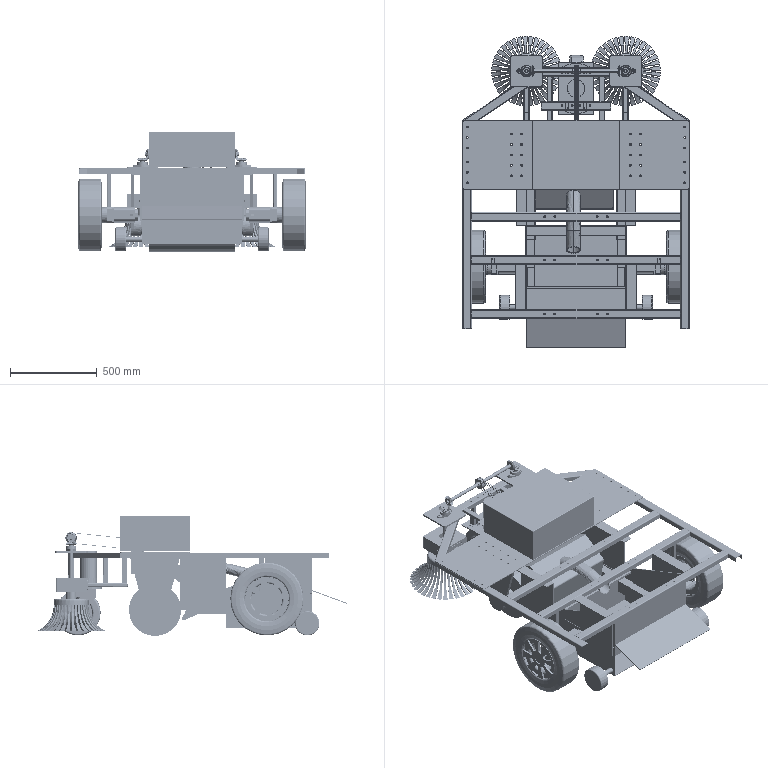Assembly | SolidWorks | mm | 97 component files | 112 solids | 5855 faces | box 1311.42 x 1789.13 x 690 mm | volume 111930544 mm3 | plane 2764 | cylinder 2030 | spline 471 | cone 310 | torus 276 | sphere 4 | commonest cylinder face diameters 10 x469 6 x221 2 x208 4 x158 8 x88 20 x80 1 x65 5 x37
Bill of materials:
50x30x2ColdBentEqualAngleSteel1000mm | 2 |  | Long, slender U-channel (formed-sheet-style profile) with a row of small round holes through the web near one end.
50x30x2ColdBentEqualAngleSteel1200mm | 4 |  | Long, slender U-channel with two pairs of small round holes in the web near the middle of its length.
50x30x2ColdBentEqualAngleSteel400 | 2 |  | Shorter U-channel with four round holes in the web and a rectangular window cut through each side flange near each end.
50x30x2ColdBentEqualAngleSteel500mm | 1 |  | Long bent strip with an angle-like profile: a flat web with a bent flange along its length and short offset or tab sections at the ends.
50x30x2ColdBentEqualAngleSteel550mmRight | 1 |  | Thin square plate with rounded corners and one central round hole. Some views also show a long, narrow channel-like strip attached to or overlapping the plate.
A30x20x2RectangularColdBentHollowSectionSteel175mm | 6 |  | Straight length of hollow rectangular tube with rounded corners, open at both ends.
A30x20x2RectangularColdFormedHollowSectionSteel220 | 2 |  | Straight length of hollow rectangular tube with rounded corners, open at both ends. It closely resembles the previous tube part.
A30x20x2RectangularColdFormedHollowSectionSteel250mm | 2 |  | Straight hollow rectangular tube with rounded corners, shown lying horizontally. The section is wider than it is tall.
Belt | 3 |  | Very thin-walled closed loop shaped like an elongated obround (stadium), similar to a band or strip loop.
BevelGear32x2 | 4 |  | Straight-tooth bevel gear with a central round bore and a single keyway.
BrushRoller | 1 |  | Stepped solid cylinder: a large-diameter central body with a smaller coaxial journal or stub shaft at each end, similar to a roller.
BrushRollerHolder | 2 |  | Hanger-type bracket: a rectangular flat top plate with a 2x5 pattern of holes, a single tapered web plate hanging below it, and a short cylindrical sleeve at the narrow lower end.
CBTCB-204.stp | 2 |  | Two-hole diamond-shaped flange with a raised round housing in the middle. A smaller cylindrical collar with a through-bore sticks up from the housing, and the collar has small radial holes.
30x20x2RectangularColdBentHollowSectionSteel900MM | 1 |  | Long straight hollow tube with a rectangular cross-section and rounded corners. One face has four small round holes, arranged as two pairs near each end.
A30x20x2RectangularColdFormedHollowSectionSteel300mm | 2 |  | Straight hollow rectangular tube fixed square to a flat rectangular plate. The plate has rounded corners and four corner holes, and the tube's opening passes through the plate.
CleaningBrush | 2 |  | Rotationally symmetric part. A small cylindrical pin with a central hole sits on top of a round hub. Many thin strip-like segments flare outward and downward from the hub in a bell or skirt shape.
CleaningBrushFixingPlate | 2 |  | Thin-walled U-shaped bracket. The flat rectangular base has four holes. Two upright side flanges are tapered, roughly triangular with a rounded tip, and each has three holes.
FixingBlock | 2 |  | Square block with rounded vertical corners. A stepped round bore goes all the way through it: a larger counterbore at the top and a smaller through-hole below. Small holes are visible on one side face.
RectangularTubeKit | 2 |  | Solid block shaped like an L (90-degree elbow), with a uniform rectangular cross-section and rounded or chamfered edges.
DriveAxis | 1 |  | Plain cylindrical shaft with chamfered ends. A short rounded-end slot (keyway) is cut into the surface near each end, both on the same side.
DriveShaft | 2 |  | Plain solid cylindrical rod or pin with flat ends and no visible features.
DriveWheel | 1 |  | Grooved wheel with three V-section grooves around its circumference. The centre bore has a keyway, and there is a recessed hub area on the face.
DSEM-GDCServoGearMotor | 1 |  | Plain cylindrical body. A small boss and a narrow shaft stick out from one end face, and the shaft has a small flat or slot.
FrontWheel | 1 |  | Wheel with a rounded tyre-like outer rim, a recessed inner face and a central hub with a small bore. Thin radial spokes or ribs connect the hub to the rim.
FrontWheelAccessory1 | 1 |  | Flat rectangular plate with a second thin layer on top that has one curved (arc) edge. A short cylindrical boss with a central hole sits on top, and small through-holes are spread across the plate.
FrontWheelAccessory2 | 1 |  | Circular disc cap with a shallow raised rim on top. Two parallel flat tabs extend down from its underside, angled to one side, and each tab ends in a rounded tip with a round hole.
GearedMotor | 1 |  | Detailed model that looks like an electric motor joined to a right-angle gearbox housing. It has a ribbed cylindrical body, a rectangular box on top with a cylindrical side spigot, a domed end cover, and a ribbed housing at the far end with a hollow bore that has a keyway.
Guard | 1 |  | Plain solid rectangular block with no visible holes or other features.
Hub | 2 |  | Spool or reel shape: a hollow cylindrical drum with a flange at each end. Inside, a spoked web has 8 openings and a small central hole.
MotorFixingPlate | 1 |  | Long, thin rectangular plate with slightly rounded corners and many small through-holes: a row along each short edge and two groups of holes in the interior.
MotorMount | 2 |  | Bent sheet-like bracket with a C-shaped profile and unequal flanges. The short top flange has 4 holes. The vertical web has a large central hole surrounded by 6 small holes on a circle. The longer bottom flange is plain.
MotorPulley1 | 1 |  | Plain cylindrical tube or spacer with a concentric through-bore and flat ends.
MotorReducer | 2 |  | Looks like a gearhead or reducer: a square front flange with 4 corner holes, a protruding round shaft, a stepped cylindrical body, and a square rear block with chamfered corners, a circular recess and a central bore.
MotorTireMotor | 2 |  | Looks like a motor body: square cross-section with cut-away corner channels, a square front flange with rounded corners and 4 holes, a round output shaft, a cylindrical rear cap, and a small block-like bump near the rear underside.
Poly-VPulley | 1 |  | Multi-groove pulley with 3 V-shaped grooves on the rim, a cylindrical hub sticking out on both sides, a central bore, a recessed face, and a small radial hole in the hub.
PushPlate | 1 |  | Thin flat rectangular plate or strip with no holes or other features.
SuctionPort | 1 |  | Prismatic block whose end profile is an irregular polygon with one large concave circular-arc edge. A bent, hollow round tube is attached to one face.
SynchronousAxis | 1 |  | Long, slender cylindrical rod with a small flat or notch near each end.
Telescopic1 | 2 |  | Straight thin-walled rectangular hollow tube with open ends.
Telescopic2 | 2 |  | Straight rectangular hollow tube with open ends and a noticeably thicker wall than a thin-gauge section.
Telescopic3 | 2 |  | Solid straight rectangular bar (a plain cuboid).
ThreadedConnectionPlate | 12 |  | L-shaped bent sheet bracket with one round through-hole in each leg.
Tire | 2 |  | Annular ring with rounded outer edges and a stepped or recessed inner face around the bore.
TorqueMotor | 2 |  | Body made of a square-section prism and a coaxial cylindrical section, with a small cylindrical shaft sticking out of the cylindrical end.
TrackPlate | 4 |  | Thin flat panel with a short bent flange along its top edge and a narrow raised line or bead across its face near the bottom.
TrashCan | 1 |  | Open-top sheet-metal box or tray with a sloped top edge on its sidewalls and rectangular cutouts. A round rod passes through it and sticks out on both sides.
TrashCanDoor | 1 |  | Thin, flat, plain rectangular plate.
TrashCanWheel | 2 |  | Thick cylindrical disc with a small central through-hole and rounded or chamfered edges.
Mates:
1. distance | 50x30x2ColdBentEqualAngleSteel1200mm-1 face at (625.629, -247.9, 410) dir (0, 1, 0) | 50x30x2ColdBentEqualAngleSteel400-1 face at (225.629, 52.1, 410) dir (0, 1, 0)
2. coincident | 50x30x2ColdBentEqualAngleSteel400-1 face at (225.629, 7.1, 415) dir (0, 0, 1) | 50x30x2ColdBentEqualAngleSteel1200mm-1 face at (625.629, -292.9, 415) dir (0, 0, 1)
3. coincident | 50x30x2ColdBentEqualAngleSteel1200mm-1 face at (-574.371, -252.9, 410) dir (-1, 0, 0) | 50x30x2ColdBentEqualAngleSteel1000mm-1 face at (-574.371, -1447.9, 410) dir (1, 0, 0)
4. coincident | 50x30x2ColdBentEqualAngleSteel1200mm-1 face at (625.629, -292.9, 415) dir (0, 0, 1) | 50x30x2ColdBentEqualAngleSteel1000mm-1 face at (-619.371, -1447.9, 415) dir (0, 0, 1)
5. coincident | 50x30x2ColdBentEqualAngleSteel1200mm-1 face at (625.629, -247.9, 410) dir (0, 1, 0) | 50x30x2ColdBentEqualAngleSteel1000mm-1 face at (-579.371, -247.9, 410) dir (0, 1, 0)
6. coincident | 50x30x2ColdBentEqualAngleSteel1200mm-1 face at (625.629, -252.9, 410) dir (1, 0, 0) | 50x30x2ColdBentEqualAngleSteel1000mm-2 face at (625.629, -1447.9, 410) dir (-1, 0, 0)
7. coincident | 50x30x2ColdBentEqualAngleSteel1200mm-1 face at (625.629, -292.9, 415) dir (0, 0, 1) | 50x30x2ColdBentEqualAngleSteel1000mm-2 face at (630.629, -1447.9, 415) dir (0, 0, 1)
8. coincident | 50x30x2ColdBentEqualAngleSteel1200mm-1 face at (625.629, -247.9, 410) dir (0, 1, 0) | 50x30x2ColdBentEqualAngleSteel1000mm-2 face at (670.629, -247.9, 410) dir (0, 1, 0)
9. coincident | 50x30x2ColdBentEqualAngleSteel400-1 face at (225.629, 7.1, 415) dir (0, 0, 1) | 50x30x2ColdBentEqualAngleSteel500mm-1 face at (-149.409, 14.658, 415) dir (0, 0, 1)
10. coincident | 50x30x2ColdBentEqualAngleSteel1000mm-1 edge at (-624.371, -247.9, 410) dir (0, 0, -1) | 50x30x2ColdBentEqualAngleSteel500mm-1 face at (-174.371, 52.1, 410) dir (-0.5547, 0.8321, 0)
11. parallel | 50x30x2ColdBentEqualAngleSteel1200mm-1 face at (625.629, -292.9, 415) dir (0, 0, 1) | CleaningRobotAssembly-1/30x20x2RectangularColdBentHollowSectionSteel900MM-2 face at (-274.371, -272.9, 238) dir (0, 0, 1)
12. coincident | 50x30x2ColdBentEqualAngleSteel400-1 edge at (-174.371, 52.1, 385) dir (0, 0, 1) | 50x30x2ColdBentEqualAngleSteel500mm-1 edge at (-174.371, 52.1, 385) dir (0, 0, 1)
13. coincident | 50x30x2ColdBentEqualAngleSteel500mm-1 face at (-149.409, 14.658, 415) dir (0, 0, 1) | 50x30x2ColdBentEqualAngleSteel550mmRight-1 face at (658.295, -290.428, 415) dir (0, 0, 1)
14. coincident | 50x30x2ColdBentEqualAngleSteel1000mm-2 edge at (675.629, -247.9, 385) dir (0, 0, 1) | 50x30x2ColdBentEqualAngleSteel550mmRight-1 face at (683.257, -252.985, 410) dir (0.5547, 0.8321, 0)
15. coincident | 50x30x2ColdBentEqualAngleSteel400-1 edge at (225.629, 52.1, 385) dir (0, 0, 1) | 50x30x2ColdBentEqualAngleSteel550mmRight-1 edge at (225.629, 52.1, 385) dir (0, 0, 1)
16. parallel | 50x30x2ColdBentEqualAngleSteel400-1 face at (225.629, 7.1, 413) dir (0, 0, -1) | FrontWheelAssembly-1/FrontWheelAccessory1-1 face at (25.629, -64.9, 238) dir (0, 0, 1)
17. parallel | 50x30x2ColdBentEqualAngleSteel400-1 face at (225.629, 7.1, 415) dir (0, 0, 1) | FrontWheelAssembly-1/FrontWheelAccessory1-1 face at (25.629, -64.9, 238) dir (0, 0, 1)
18. concentric | FrontWheelAssembly-1/FrontWheelAccessory1-1 face at (25.629, -64.9, 235) dir (0, 0, 1) r 10 | DSEM-GDCServoGearMotor-1 face at (25.629, -64.9, 232.831) dir (0, 0, -1) r 7
19. coincident | FrontWheelAssembly-1/FrontWheelAccessory1-1 face at (25.629, -64.9, 268) dir (0, 0, 1) | DSEM-GDCServoGearMotor-1 face at (44.794, -59.181, 268) dir (0, 0, -1)
20. parallel | 50x30x2ColdBentEqualAngleSteel1000mm-1 face at (-624.371, -1447.9, 410) dir (-1, 0, 0) | FrontWheelAssembly-1/FrontWheelAccessory1-1 face at (-74.371, -214.9, 233) dir (-1, 0, 0)
21. coincident | 50x30x2ColdBentEqualAngleSteel400-1 face at (225.629, 7.1, 413) dir (0, 0, -1) | A30x20x2RectangularColdBentHollowSectionSteel175mm-1 face at (76.629, 35.1, 413) dir (0, 0, 1)
22. parallel | 50x30x2ColdBentEqualAngleSteel400-1 face at (225.629, 52.1, 410) dir (0, 1, 0) | A30x20x2RectangularColdBentHollowSectionSteel175mm-1 face at (76.629, 50.1, 238) dir (0, 1, 0)
23. coincident | 50x30x2ColdBentEqualAngleSteel400-1 face at (225.629, 50.1, 410) dir (0, -1, 0) | A30x20x2RectangularColdBentHollowSectionSteel175mm-1 face at (76.629, 50.1, 238) dir (0, 1, 0)
24. coincident | FrontWheelAssembly-1/FrontWheelAccessory1-1 face at (25.629, -64.9, 238) dir (0, 0, 1) | A30x20x2RectangularColdBentHollowSectionSteel175mm-1 face at (76.629, 35.1, 238) dir (0, 0, -1)
25. coincident | FrontWheelAssembly-1/FrontWheelAccessory1-1 face at (25.629, -64.9, 238) dir (0, 0, 1) | ThreadedConnectionPlate-1 face at (102.629, 35.1, 238) dir (0, 0, -1)
26. coincident | A30x20x2RectangularColdBentHollowSectionSteel175mm-1 face at (86.629, 35.1, 238) dir (1, 0, 0) | ThreadedConnectionPlate-1 face at (86.629, 35.1, 238) dir (-1, 0, 0)
27. coincident | A30x20x2RectangularColdBentHollowSectionSteel175mm-1 face at (76.629, 50.1, 238) dir (0, 1, 0) | ThreadedConnectionPlate-1 face at (117.629, 50.1, 239) dir (0, 1, 0)
28. concentric | FrontWheelAssembly-1/FrontWheelAccessory1-1 face at (105.629, 35.1, 238) dir (0, 0, -1) r 5 | ThreadedConnectionPlate-1 face at (105.629, 35.1, 238) dir (0, 0, 1) r 5
29. coincident | A30x20x2RectangularColdBentHollowSectionSteel175mm-1 face at (66.629, 35.1, 238) dir (-1, 0, 0) | ThreadedConnectionPlate-6 face at (66.629, 35.1, 238) dir (1, 0, 0)
30. coincident | A30x20x2RectangularColdBentHollowSectionSteel175mm-1 face at (76.629, 50.1, 238) dir (0, 1, 0) | ThreadedConnectionPlate-6 face at (35.629, 50.1, 239) dir (0, 1, 0)
31. coincident | FrontWheelAssembly-1/FrontWheelAccessory1-1 face at (25.629, -64.9, 238) dir (0, 0, 1) | ThreadedConnectionPlate-6 face at (50.629, 35.1, 238) dir (0, 0, -1)
32. coincident | 50x30x2ColdBentEqualAngleSteel400-1 face at (225.629, 7.1, 413) dir (0, 0, -1) | A30x20x2RectangularColdBentHollowSectionSteel175mm-4 face at (-25.371, 35.1, 413) dir (0, 0, 1)
33. coincident | 50x30x2ColdBentEqualAngleSteel400-1 face at (225.629, 50.1, 410) dir (0, -1, 0) | A30x20x2RectangularColdBentHollowSectionSteel175mm-4 face at (-25.371, 50.1, 238) dir (0, 1, 0)
34. coincident | FrontWheelAssembly-1/FrontWheelAccessory1-1 face at (25.629, -64.9, 238) dir (0, 0, 1) | ThreadedConnectionPlate-10 face at (0.6293, 35.1, 238) dir (0, 0, -1)
35. coincident | ThreadedConnectionPlate-10 face at (-15.371, 35.1, 238) dir (-1, 0, 0) | A30x20x2RectangularColdBentHollowSectionSteel175mm-4 face at (-15.371, 35.1, 238) dir (1, 0, 0)
36. concentric | FrontWheelAssembly-1/FrontWheelAccessory1-1 face at (3.629, 35.1, 253) dir (0, 0, -1) r 5.507 | ThreadedConnectionPlate-10 face at (3.629, 35.1, 238) dir (0, 0, 1) r 5
37. concentric | FrontWheelAssembly-1/FrontWheelAccessory1-1 face at (-54.371, 35.1, 238) dir (0, 0, -1) r 5 | ThreadedConnectionPlate-8 face at (-54.371, 35.1, 238) dir (0, 0, 1) r 5
38. coincident | FrontWheelAssembly-1/FrontWheelAccessory1-1 face at (25.629, -64.9, 238) dir (0, 0, 1) | ThreadedConnectionPlate-8 face at (-51.371, 35.1, 238) dir (0, 0, -1)
39. coincident | ThreadedConnectionPlate-8 face at (-35.371, 35.1, 238) dir (1, 0, 0) | A30x20x2RectangularColdBentHollowSectionSteel175mm-4 face at (-35.371, 35.1, 238) dir (-1, 0, 0)
40. coincident | A30x20x2RectangularColdBentHollowSectionSteel175mm-3 face at (76.629, -164.9, 413) dir (0, 0, 1) | 50x30x2ColdBentEqualAngleSteel400-2 face at (225.629, -184.9, 413) dir (0, 0, -1)
41. coincident | 50x30x2ColdBentEqualAngleSteel400-1 face at (-174.371, 47.1, 410) dir (-1, 0, 0) | 50x30x2ColdBentEqualAngleSteel400-2 face at (-174.371, -144.9, 410) dir (-1, 0, 0)
42. coincident | 50x30x2ColdBentEqualAngleSteel1200mm-1 face at (625.629, -247.9, 410) dir (0, 1, 0) | A30x20x2RectangularColdFormedHollowSectionSteel250mm-1 face at (-124.591, -247.9, 400) dir (0, -1, 0)
43. distance | A30x20x2RectangularColdFormedHollowSectionSteel250mm-1 face at (-124.591, -247.9, 410) dir (0, 0, 1) | 50x30x2ColdBentEqualAngleSteel400-1 face at (225.629, 7.1, 415) dir (0, 0, 1)
44. coincident | 50x30x2ColdBentEqualAngleSteel400-1 face at (185.629, -14.9, 410) dir (0, 0, -1) | A30x20x2RectangularColdFormedHollowSectionSteel250mm-2 face at (175.629, -247.9, 410) dir (0, 0, 1)
45. coincident | 50x30x2ColdBentEqualAngleSteel400-1 face at (160.629, -14.9, 395) dir (1, 0, 0) | A30x20x2RectangularColdFormedHollowSectionSteel250mm-2 face at (160.629, -247.9, 400) dir (-1, 0, 0)
46. coincident | 50x30x2ColdBentEqualAngleSteel400-1 face at (225.629, 52.1, 410) dir (0, 1, 0) | A30x20x2RectangularColdFormedHollowSectionSteel250mm-2 face at (175.629, 52.1, 400) dir (0, 1, 0)
47. concentric | FrontWheelAssembly-1/FrontWheelAccessory1-1 face at (-54.371, -164.9, 144) dir (0, 0, 1) r 5 | 50x30x2ColdBentEqualAngleSteel400-2 face at (-54.371, -164.9, 350) dir (0, 0, 1) r 5
48. coincident | CleaningRobotAssembly-1/30x20x2RectangularColdBentHollowSectionSteel900MM-2 face at (-274.371, -272.9, 238) dir (0, 0, 1) | A30x20x2RectangularColdBentHollowSectionSteel175mm-6 face at (176.629, -272.9, 238) dir (0, 0, -1)
49. coincident | 50x30x2ColdBentEqualAngleSteel1200mm-1 face at (625.629, -292.9, 413) dir (0, 0, -1) | A30x20x2RectangularColdBentHollowSectionSteel175mm-6 face at (176.629, -272.9, 413) dir (0, 0, 1)
50. coincident | A30x20x2RectangularColdBentHollowSectionSteel175mm-6 face at (186.629, -272.9, 238) dir (1, 0, 0) | ThreadedConnectionPlate-12 face at (186.629, -272.9, 238) dir (-1, 0, 0)
51. coincident | A30x20x2RectangularColdBentHollowSectionSteel175mm-6 face at (176.629, -287.9, 238) dir (0, -1, 0) | ThreadedConnectionPlate-12 face at (217.629, -287.9, 239) dir (0, -1, 0)
52. concentric | CleaningRobotAssembly-1/30x20x2RectangularColdBentHollowSectionSteel900MM-2 face at (205.629, -272.9, 301) dir (0, 0, -1) r 5 | ThreadedConnectionPlate-12 face at (205.629, -272.9, 238) dir (0, 0, 1) r 5
53. coincident | CleaningRobotAssembly-1/30x20x2RectangularColdBentHollowSectionSteel900MM-2 face at (-274.371, -272.9, 238) dir (0, 0, 1) | ThreadedConnectionPlate-12 face at (202.629, -272.9, 238) dir (0, 0, -1)
54. concentric | CleaningRobotAssembly-1/30x20x2RectangularColdBentHollowSectionSteel900MM-2 face at (147.629, -272.9, 301) dir (0, 0, -1) r 5 | ThreadedConnectionPlate-13 face at (147.629, -272.9, 238) dir (0, 0, 1) r 5
55. coincident | CleaningRobotAssembly-1/30x20x2RectangularColdBentHollowSectionSteel900MM-2 face at (-274.371, -272.9, 238) dir (0, 0, 1) | ThreadedConnectionPlate-13 face at (150.629, -272.9, 238) dir (0, 0, -1)
56. coincident | A30x20x2RectangularColdBentHollowSectionSteel175mm-6 face at (166.629, -272.9, 238) dir (-1, 0, 0) | ThreadedConnectionPlate-13 face at (166.629, -272.9, 238) dir (1, 0, 0)
57. coincident | 50x30x2ColdBentEqualAngleSteel1000mm-1 face at (-624.371, -1447.9, 410) dir (-1, 0, 0) | MotorFixingPlate-1 face at (-624.371, -647.9, 420) dir (-1, 0, 0)
58. coincident | 50x30x2ColdBentEqualAngleSteel1000mm-1 face at (-619.371, -1447.9, 415) dir (0, 0, 1) | MotorFixingPlate-1 face at (25.629, -447.9, 415) dir (0, 0, -1)
59. parallel | MotorFixingPlate-1 face at (25.629, -447.9, 415) dir (0, 0, -1) | TorqueMotor-1 face at (-92.371, -325.407, 376) dir (0, 0, 1)
60. concentric | BrushRoller-1 face at (-324.371, -447.9, 85) dir (1, 0, 0) r 50 | BrushRollerHolder-1 face at (-308.371, -447.9, 85) dir (-1, 0, 0) r 50
61. coincident | MotorFixingPlate-1 face at (25.629, -447.9, 415) dir (0, 0, -1) | BrushRollerHolder-1 face at (-316.371, -447.9, 415) dir (0, 0, 1)
62. concentric | MotorFixingPlate-1 face at (-345.371, -567.9, 380) dir (0, 0, 1) r 5 | BrushRollerHolder-1 face at (-345.371, -567.9, 450) dir (0, 0, -1) r 5
63. coincident | MotorFixingPlate-1 face at (25.629, -447.9, 415) dir (0, 0, -1) | MotorMount-1 face at (-227.371, -367.407, 415) dir (0, 0, 1)
64. concentric | TorqueMotor-1 face at (-224.371, -367.407, 334) dir (1, 0, 0) r 37 | MotorMount-1 face at (-248.371, -367.407, 334) dir (1, 0, 0) r 20
65. concentric | TorqueMotor-1 face at (-214.371, -367.407, 364) dir (-1, 0, 0) r 3 | MotorMount-1 face at (-224.371, -367.407, 364) dir (-1, 0, 0) r 3
66. coincident | TorqueMotor-1 face at (-224.371, -367.407, 334) dir (-1, 0, 0) | MotorMount-1 face at (-224.371, -367.407, 334) dir (1, 0, 0)
67. concentric | MotorFixingPlate-1 face at (-287.371, -567.9, 380) dir (0, 0, 1) r 5 | BrushRollerHolder-1 face at (-287.371, -567.9, 450) dir (0, 0, -1) r 5
68. concentric | TorqueMotor-1 face at (-254.371, -367.407, 334) dir (1, 0, 0) r 8 | MotorPulley1-1 face at (-234.371, -367.407, 334) dir (-1, 0, 0) r 8
69. coincident | TorqueMotor-1 face at (-254.371, -367.407, 334) dir (-1, 0, 0) | MotorPulley1-1 face at (-254.371, -367.407, 334) dir (-1, 0, 0)
70. concentric | MotorTireMotor-1 face at (-468.371, -1090.9, 148) dir (1, 0, 0) r 11 | MotorReducer-1 face at (-470.371, -1090.9, 148) dir (1, 0, 0) r 11
71. coincident | MotorTireMotor-1 face at (-434.371, -1090.9, 148) dir (-1, 0, 0) | MotorReducer-1 face at (-434.371, -1090.9, 148) dir (1, 0, 0)
72. coincident | MotorTireMotor-1 face at (-422.371, -1045.9, 193) dir (0, 0, 1) | MotorReducer-1 face at (-462.371, -1135.9, 193) dir (0, 0, 1)
73. concentric | Hub-1 face at (-621.371, -1090.9, 148) dir (-1, 0, 0) r 93 | Tire-1 face at (-664.825, -1090.9, 148) dir (-1, 0, 0) r 108
74. coincident | Hub-1 face at (-608.371, -1009.58, 206.198) dir (1, 0, 0) | Tire-1 face at (-608.371, -983.391, 137.711) dir (-1, 0, 0)
75. concentric | Hub-1 face at (-501.371, -1090.9, 148) dir (-1, 0, 0) r 10 | MotorReducer-1 face at (-619.371, -1090.9, 148) dir (1, 0, 0) r 10
76. coincident | Hub-1 face at (-619.371, -1090.9, 148) dir (-1, 0, 0) | MotorReducer-1 face at (-619.371, -1090.9, 148) dir (-1, 0, 0)
77. coincident | 50x30x2ColdBentEqualAngleSteel1000mm-1 face at (-574.371, -1447.9, 410) dir (1, 0, 0) | 50x30x2ColdBentEqualAngleSteel1200mm-2 face at (-574.371, -1032.9, 410) dir (-1, 0, 0)
78. coincident | 50x30x2ColdBentEqualAngleSteel1000mm-1 face at (-619.371, -1447.9, 415) dir (0, 0, 1) | 50x30x2ColdBentEqualAngleSteel1200mm-2 face at (625.629, -1072.9, 415) dir (0, 0, 1)
79. parallel | MotorTireMotor-1 face at (-422.371, -1045.9, 193) dir (0, 0, 1) | 50x30x2ColdBentEqualAngleSteel1200mm-2 face at (625.629, -1072.9, 413) dir (0, 0, -1)
80. coincident | 50x30x2ColdBentEqualAngleSteel1200mm-2 face at (625.629, -1072.9, 413) dir (0, 0, -1) | A30x20x2RectangularColdFormedHollowSectionSteel220-1 face at (-452.371, -1060.9, 413) dir (0, 0, 1)
81. coincident | MotorReducer-1 face at (-462.371, -1135.9, 193) dir (0, 0, 1) | A30x20x2RectangularColdFormedHollowSectionSteel220-1 face at (-452.371, -1060.9, 193) dir (0, 0, -1)
82. coincident | 50x30x2ColdBentEqualAngleSteel1200mm-2 face at (625.629, -1075.9, 410) dir (0, 1, 0) | A30x20x2RectangularColdFormedHollowSectionSteel220-1 face at (-452.371, -1075.9, 413) dir (0, -1, 0)
83. coincident | MotorReducer-1 face at (-462.371, -1045.9, 103) dir (0, 1, 0) | A30x20x2RectangularColdFormedHollowSectionSteel220-1 face at (-452.371, -1045.9, 413) dir (0, 1, 0)
84. parallel | 50x30x2ColdBentEqualAngleSteel1000mm-1 face at (-579.371, -1447.9, 410) dir (0, -1, 0) | TrashCan-1 face at (-264.371, -1353.331, 103.161) dir (0, -1, 0)
85. coincident | BrushRoller-1 face at (-324.371, -447.9, 85) dir (-1, 0, 0) | BrushRollerHolder-1 face at (-324.371, -447.9, 85) dir (-1, 0, 0)
86. parallel | BrushRollerHolder-1 face at (-324.371, -447.9, 85) dir (-1, 0, 0) | MotorMount-1 face at (-227.371, -367.407, 334) dir (-1, 0, 0)
87. coincident | BrushRoller-1 face at (-224.371, -447.9, 85) dir (-1, 0, 0) | TorqueMotor-1 face at (-224.371, -367.407, 334) dir (-1, 0, 0)
88. coincident | 50x30x2ColdBentEqualAngleSteel1200mm-1 face at (625.629, -247.9, 410) dir (0, 1, 0) | MotorFixingPlate-1 face at (-624.371, -247.9, 420) dir (0, 1, 0)
89. concentric | MotorFixingPlate-1 face at (-212.371, -407.407, 895) dir (0, 0, -1) r 5 | MotorMount-1 face at (-212.371, -407.407, 412) dir (0, 0, 1) r 5
90. concentric | MotorFixingPlate-1 face at (-212.371, -327.407, 895) dir (0, 0, -1) r 5 | MotorMount-1 face at (-212.371, -327.407, 412) dir (0, 0, 1) r 5
91. coincident | 50x30x2ColdBentEqualAngleSteel1000mm-1 face at (-574.371, -1447.9, 410) dir (1, 0, 0) | 50x30x2ColdBentEqualAngleSteel1200mm-3 face at (-574.371, -1342.9, 410) dir (-1, 0, 0)
92. coincident | 50x30x2ColdBentEqualAngleSteel1000mm-1 face at (-619.371, -1447.9, 415) dir (0, 0, 1) | 50x30x2ColdBentEqualAngleSteel1200mm-3 face at (625.629, -1382.9, 415) dir (0, 0, 1)
93. distance | 50x30x2ColdBentEqualAngleSteel1200mm-2 face at (625.629, -1077.9, 410) dir (0, -1, 0) | 50x30x2ColdBentEqualAngleSteel1200mm-3 face at (625.629, -1337.9, 410) dir (0, 1, 0)
94. coincident | 50x30x2ColdBentEqualAngleSteel1000mm-1 face at (-624.371, -1447.9, 410) dir (-1, 0, 0) | Hub-1 face at (-624.371, -1090.9, 148) dir (-1, 0, 0)
95. coincident | MotorReducer-1 face at (-462.371, -1090.9, 148) dir (-1, 0, 0) | A30x20x2RectangularColdFormedHollowSectionSteel220-1 face at (-462.371, -1060.9, 413) dir (-1, 0, 0)
96. coincident | TrashCan-1 face at (-264.371, -1353.331, -21.839) dir (-1, 0, 0) | TrackPlate-1 face at (-264.371, -1337.9, 410) dir (1, 0, 0)
97. coincident | 50x30x2ColdBentEqualAngleSteel1200mm-3 face at (625.629, -1382.9, 415) dir (0, 0, 1) | TrackPlate-1 face at (-294.371, -1207.9, 415) dir (0, 0, 1)
98. coincident | 50x30x2ColdBentEqualAngleSteel1200mm-2 face at (625.629, -1077.9, 410) dir (0, -1, 0) | TrackPlate-1 face at (-264.371, -1077.9, 410) dir (0, 1, 0)
99. distance | 50x30x2ColdBentEqualAngleSteel1200mm-3 face at (625.629, -1387.9, 410) dir (0, -1, 0) | 50x30x2ColdBentEqualAngleSteel1000mm-1 face at (-579.371, -1447.9, 410) dir (0, -1, 0)
100. coincident | 50x30x2ColdBentEqualAngleSteel1200mm-2 face at (625.629, -1077.9, 410) dir (0, -1, 0) | TrackPlate-2 face at (315.629, -1077.9, 410) dir (0, 1, 0)
101. coincident | 50x30x2ColdBentEqualAngleSteel1200mm-2 face at (625.629, -1072.9, 415) dir (0, 0, 1) | TrackPlate-2 face at (345.629, -1207.9, 415) dir (0, 0, 1)
102. coincident | TrashCan-1 face at (315.629, -1353.331, -21.839) dir (1, 0, 0) | TrackPlate-2 face at (315.629, -1077.9, 410) dir (-1, 0, 0)
103. concentric | TrashCan-1 face at (-264.371, -939.331, 178.161) dir (0, -1, 0) r 2.5 | TrackPlate-1 face at (-264.371, -1070.829, 178.161) dir (0, -1, 0) r 2.5
104. parallel | 50x30x2ColdBentEqualAngleSteel1200mm-1 face at (625.629, -297.9, 410) dir (0, -1, 0) | CleaningRobotAssembly-1/RectangularTubeKit-1 face at (322.629, -289.9, 221) dir (0, -1, 0)
105. concentric | 50x30x2ColdBentEqualAngleSteel1200mm-1 face at (-154.371, -272.9, 405) dir (0, 0, 1) r 5 | CleaningRobotAssembly-1/30x20x2RectangularColdBentHollowSectionSteel900MM-2 face at (-154.371, -272.9, 301) dir (0, 0, -1) r 5
106. distance | TrackPlate-1 face at (-264.371, -1337.9, 410) dir (1, 0, 0) | 50x30x2ColdBentEqualAngleSteel1000mm-1 face at (-574.371, -1447.9, 410) dir (1, 0, 0)
107. concentric | TrashCan-1 face at (-414.371, -1323.331, 8.161) dir (1, 0, 0) r 15 | TrashCanWheel-3 face at (-414.371, -1323.331, 8.161) dir (1, 0, 0) r 15
108. coincident | TrashCan-1 face at (-414.371, -1323.331, 8.161) dir (-1, 0, 0) | TrashCanWheel-3 face at (-414.371, -1323.331, 8.161) dir (-1, 0, 0)
109. concentric | TrashCan-1 face at (465.629, -1323.331, 8.161) dir (-1, 0, 0) r 15 | TrashCanWheel-4 face at (405.629, -1323.331, 8.161) dir (1, 0, 0) r 15
110. coincident | TrashCan-1 face at (465.629, -1323.331, 8.161) dir (1, 0, 0) | TrashCanWheel-4 face at (465.629, -1323.331, 8.161) dir (1, 0, 0)
111. distance | SuctionPort-1 face at (240.629, -545.604, 83.86) dir (1, 0, 0) | TrashCan-1 face at (315.629, -1353.331, -21.839) dir (1, 0, 0)
112. coincident | SuctionPort-1 face at (-209.371, -545.604, 83.86) dir (-1, 0, 0) | Telescopic1-1 face at (-209.371, -636.122, 139.31) dir (1, 0, 0)
113. parallel | CleaningRobotAssembly-1/CleaningBrushFixingPlate-3 face at (-350.371, -57.9, 188) dir (0, -1, 0) | Telescopic1-1 face at (-234.371, -636.122, 101.81) dir (0, 1, 0)
114. coincident | Telescopic1-1 face at (-257.371, -436.122, 67.31) dir (0, 0, 1) | Telescopic2-1 face at (-257.371, -793.365, 67.31) dir (0, 0, -1)
115. coincident | Telescopic1-1 face at (-257.371, -436.122, 67.31) dir (1, 0, 0) | Telescopic2-1 face at (-257.371, -793.365, 67.31) dir (-1, 0, 0)
116. coincident | TrashCan-1 face at (-264.371, -1230.322, -16.839) dir (0, 0, 1) | PushPlate-1 face at (-259.371, -1216.787, -16.839) dir (0, 0, -1)
117. coincident | TrashCan-1 face at (310.629, -1353.331, -21.839) dir (-1, 0, 0) | PushPlate-1 face at (310.629, -1216.787, -16.839) dir (1, 0, 0)
118. coincident | Telescopic2-1 face at (-254.371, -1093.365, 72.31) dir (1, 0, 0) | Telescopic3-1 face at (-254.371, -906.787, 72.31) dir (-1, 0, 0)
119. coincident | Telescopic2-1 face at (-254.371, -1093.365, 72.31) dir (0, 0, 1) | Telescopic3-1 face at (-254.371, -906.787, 72.31) dir (0, 0, -1)
120. coincident | PushPlate-1 face at (25.629, -1206.787, 90.661) dir (0, 1, 0) | Telescopic3-1 face at (-234.371, -1206.787, 102.31) dir (0, -1, 0)
121. distance | Telescopic2-1 face at (-234.371, -1093.365, 102.31) dir (0, -1, 0) | Telescopic1-1 face at (-234.371, -936.122, 101.81) dir (0, -1, 0)
122. distance | PushPlate-1 face at (25.629, -1206.787, 90.661) dir (0, 1, 0) | Telescopic2-1 face at (-234.371, -1093.365, 102.31) dir (0, -1, 0)
123. coincident | 50x30x2ColdBentEqualAngleSteel1000mm-1 face at (-574.371, -1447.9, 410) dir (1, 0, 0) | 50x30x2ColdBentEqualAngleSteel1200mm-4 face at (-574.371, -782.9, 410) dir (-1, 0, 0)
124. coincident | 50x30x2ColdBentEqualAngleSteel1000mm-1 face at (-619.371, -1447.9, 415) dir (0, 0, 1) | 50x30x2ColdBentEqualAngleSteel1200mm-4 face at (625.629, -822.9, 415) dir (0, 0, 1)
125. distance | 50x30x2ColdBentEqualAngleSteel1200mm-4 face at (625.629, -827.9, 410) dir (0, -1, 0) | 50x30x2ColdBentEqualAngleSteel1200mm-2 face at (625.629, -1027.9, 410) dir (0, 1, 0)
126. coincident | Telescopic1-1 face at (-259.371, -636.122, 139.31) dir (-1, 0, 0) | TrackPlate-3 face at (-259.371, -853.293, 380) dir (1, 0, 0)
127. coincident | 50x30x2ColdBentEqualAngleSteel1200mm-4 face at (625.629, -777.9, 385) dir (0, 0, -1) | TrackPlate-3 face at (-289.371, -723.293, 385) dir (0, 0, 1)
128. coincident | TrashCan-1 face at (-259.371, -1353.331, -21.839) dir (1, 0, 0) | TrashCanDoor-1 face at (-259.371, -1351.6, 193.47) dir (-1, 0, 0)
129. coincident | TrashCan-1 edge at (310.629, -1353.331, 198.161) dir (-1, 0, 0) | TrashCanDoor-1 edge at (-259.371, -1353.331, 198.161) dir (1, 0, 0)
130. concentric | CleaningRobotAssembly-1/CleaningBrush-1 face at (310.629, 34.1, 198) dir (0, 0, 1) r 10 | CBTCB-204.stp-1 face at (310.629, 34.1, 436) dir (0, 0, 1) r 10
131. coincident | 50x30x2ColdBentEqualAngleSteel550mmRight-1 face at (197.894, 10.497, 425) dir (0, 0, 1) | CBTCB-204.stp-1 face at (265.629, 34.1, 425) dir (0, 0, -1)
132. parallel | CleaningRobotAssembly-1/FixingBlock-1 face at (400.629, 124.1, 188) dir (0, 1, 0) | CBTCB-204.stp-1 face at (355.629, 45.6, 434) dir (0, 1, 0)
133. concentric | CleaningRobotAssembly-1/FixingBlock-3 face at (-259.371, 34.1, 288) dir (0, 0, -1) r 32.5 | CBTCB-204.stp-2 face at (-259.371, 34.1, 450.5) dir (0, 0, -1) r 14
134. coincident | 50x30x2ColdBentEqualAngleSteel550mmRight-1 face at (197.894, 10.497, 425) dir (0, 0, 1) | CBTCB-204.stp-2 face at (-304.371, 34.1, 425) dir (0, 0, -1)
135. parallel | 50x30x2ColdBentEqualAngleSteel550mmRight-1 face at (-349.371, 124.019, 425) dir (0, 1, 0) | CBTCB-204.stp-2 face at (-287.079, 45.6, 434) dir (0, 1, 0)
136. concentric | CleaningRobotAssembly-1/CleaningBrush-1 face at (310.629, 34.1, 198) dir (0, 0, 1) r 10 | DriveShaft-1 face at (310.629, 34.1, 478.3) dir (0, 0, -1) r 10
137. concentric | DriveShaft-1 face at (310.629, 34.1, 478.3) dir (0, 0, -1) r 10 | BevelGear32x2-1 face at (310.629, 34.1, 459.816) dir (0, 0, 1) r 10
138. coincident | DriveShaft-1 face at (303.781, 36.187, 474.3) dir (0.6655, 0.7464, 0) | BevelGear32x2-1 face at (303.259, 36.653, 459.816) dir (0.6655, 0.7464, 0)
139. distance | DriveShaft-1 face at (310.629, 34.1, 478.3) dir (0, 0, 1) | BevelGear32x2-1 face at (294.862, 48.16, 473.836) dir (0, 0, 1)
140. distance | DriveShaft-1 face at (310.629, 34.1, 478.3) dir (0, 0, 1) | CBTCB-204.stp-1 face at (320.629, 34.1, 458.3) dir (0, 0, 1)
141. coincident | BevelGear32x2-1 sketch point at (310.629, 34.1, 498.836) dir (1, 0, 0) | BevelGear32x2-2 sketch point at (310.629, 34.1, 498.836) dir (1, 0, 0)
142. parallel | 50x30x2ColdBentEqualAngleSteel550mmRight-1 face at (400.629, 125.228, 425) dir (1, 0, 0) | BevelGear32x2-2 face at (271.61, 27.247, 495.68) dir (-1, 0, 0)
143. concentric | CBTCB-204.stp-2 face at (-259.371, 34.1, 436) dir (0, 0, 1) r 10 | DriveShaft-2 face at (-259.371, 34.1, 478.3) dir (0, 0, -1) r 10
144. coincident | DriveShaft-1 face at (310.629, 34.1, 478.3) dir (0, 0, 1) | DriveShaft-2 face at (-259.371, 34.1, 478.3) dir (0, 0, 1)
145. concentric | DriveShaft-2 face at (-259.371, 34.1, 478.3) dir (0, 0, -1) r 10 | BevelGear32x2-3 face at (-259.371, 34.1, 459.816) dir (0, 0, 1) r 10
146. distance | DriveShaft-2 face at (-259.371, 34.1, 478.3) dir (0, 0, 1) | BevelGear32x2-3 face at (-275.26, 48.022, 473.836) dir (0, 0, 1)
147. coincident | DriveShaft-2 face at (-266.237, 36.127, 474.3) dir (0.659, 0.7521, 0) | BevelGear32x2-3 face at (-266.763, 36.588, 459.816) dir (0.659, 0.7521, 0)
148. coincident | BevelGear32x2-3 sketch point at (-259.371, 34.1, 498.836) dir (1, 0, 0) | BevelGear32x2-4 sketch point at (-259.371, 34.1, 498.836) dir (1, 0, 0)
149. parallel | 50x30x2ColdBentEqualAngleSteel550mmRight-1 face at (-169.371, -55.981, 425) dir (1, 0, 0) | BevelGear32x2-4 face at (-220.351, 26.662, 497.567) dir (1, 0, 0)
150. concentric | BevelGear32x2-2 face at (271.61, 34.1, 498.836) dir (1, 0, 0) r 10 | SynchronousAxis-1 face at (295.629, 34.1, 498.836) dir (-1, 0, 0) r 10
151. width | SynchronousAxis-1 face at (295.629, 34.1, 498.836) dir (1, 0, 0) | SynchronousAxis-1 face at (-244.371, 34.1, 498.836) dir (-1, 0, 0) | BevelGear32x2-4 face at (-234.371, 13.275, 495.283) dir (-1, 0, 0) | BevelGear32x2-2 face at (285.63, 14.911, 490) dir (1, 0, 0)
152. coincident | BevelGear32x2-2 face at (271.61, 28.815, 493.099) dir (0, -0.4182, 0.9083) | SynchronousAxis-1 face at (320.629, 29.45, 493.392) dir (0, -0.4182, 0.9083)
153. coincident | MotorFixingPlate-1 face at (25.629, -447.9, 420) dir (0, 0, 1) | GearedMotor-1 face at (128.629, -385.9, 420) dir (0, 0, -1)
154. concentric | GearedMotor-1 face at (80.629, -347.9, 460) dir (1, 0, 0) r 7 | DriveWheel-1 face at (41.44, -347.9, 460) dir (-1, 0, 0) r 7
155. distance | GearedMotor-1 face at (145.629, -359.538, 448.362) dir (1, 0, 0) | 50x30x2ColdBentEqualAngleSteel1000mm-2 face at (675.629, -1447.9, 410) dir (1, 0, 0)
156. concentric | GearedMotor-1 face at (80.629, -347.9, 460) dir (1, 0, 0) r 7 | DriveAxis-1 face at (145.629, -347.9, 460) dir (-1, 0, 0) r 7
157. coincident | DriveWheel-1 face at (15.629, -347.9, 470.365) dir (-1, 0, 0) | DriveAxis-1 face at (15.629, -347.9, 460) dir (-1, 0, 0)
158. coincident | GearedMotor-1 face at (145.629, -359.538, 448.362) dir (1, 0, 0) | DriveAxis-1 face at (145.629, -347.9, 460) dir (1, 0, 0)
159. coincident | GearedMotor-1 face at (117.33, -350.4, 466.538) dir (0, 1, 0) | DriveAxis-1 face at (145.629, -350.4, 464.7) dir (0, 1, 0)
160. coincident | DriveWheel-1 face at (41.44, -345.4, 464.75) dir (0, -1, 0) | DriveAxis-1 face at (15.629, -345.4, 464.7) dir (0, -1, 0)
161. concentric | SynchronousAxis-1 face at (295.629, 34.1, 498.836) dir (-1, 0, 0) r 10 | Poly-VPulley-1 face at (15.04, 34.1, 498.836) dir (1, 0, 0) r 10
162. distance | GearedMotor-1 face at (85.129, -307.9, 470.739) dir (0, 1, 0) | 50x30x2ColdBentEqualAngleSteel1200mm-1 face at (625.629, -247.9, 410) dir (0, 1, 0)
163. distance | BevelGear32x2-4 face at (-220.351, 26.662, 497.567) dir (1, 0, 0) | Poly-VPulley-1 face at (15.04, 14.37, 497.166) dir (-1, 0, 0)
164. coincident | 50x30x2ColdBentEqualAngleSteel550mmRight-1 face at (197.894, 10.497, 425) dir (0, 0, 1) | Guard-1 face at (275.629, -647.9, 425) dir (0, 0, -1)
165. coincident | MotorFixingPlate-1 face at (-624.371, -647.9, 420) dir (0, -1, 0) | Guard-1 face at (25.629, -647.9, 625) dir (0, -1, 0)
166. distance | Guard-1 face at (275.629, -447.9, 625) dir (1, 0, 0) | 50x30x2ColdBentEqualAngleSteel1000mm-2 face at (675.629, -1447.9, 410) dir (1, 0, 0)
167. gear | BevelGear32x2-1 face at (310.629, 34.1, 459.816) dir (0, 0, 1) r 10 | BevelGear32x2-2 face at (271.61, 34.1, 498.836) dir (1, 0, 0) r 10
168. gear | BevelGear32x2-4 face at (-220.351, 34.1, 498.836) dir (-1, 0, 0) r 10 | BevelGear32x2-3 face at (-259.371, 34.1, 459.816) dir (0, 0, 1) r 10
169. concentric | CleaningBrush-1 face at (-257.138, 891.798, 90) dir (0, 1, 0) r 30 | FixingBlock-1 face at (-257.138, 765.176, 90) dir (0, 1, 0) r 32.5
170. distance | FixingBlock-1 face at (-257.138, 785.176, 90) dir (0, -1, 0) | CleaningBrush-1 face at (-236.441, 745.176, 68.282) dir (0, 1, 0)
171. concentric | CleaningBrush-1 face at (-257.138, 795.176, 90) dir (0, 1, 0) r 10 | DSEM-GDCServoGearMotor-1 face at (-257.138, 810.007, 90) dir (0, -1, 0) r 7
172. coincident | CleaningBrush-1 face at (-257.138, 845.176, 90) dir (0, 1, 0) | DSEM-GDCServoGearMotor-1 face at (-276.324, 845.176, 84.352) dir (0, -1, 0)
173. coincident | FixingBlock-1 face at (-167.138, 785.176, 0) dir (1, 0, 0) | CleaningBrushFixingPlate-1 face at (-167.138, 865.176, 180) dir (-1, 0, 0)
174. coincident | FixingBlock-1 face at (-257.138, 865.176, 90) dir (0, 1, 0) | CleaningBrushFixingPlate-1 face at (-257.138, 865.176, 180) dir (0, 1, 0)
175. coincident | FixingBlock-1 face at (-167.138, 785.176, 180) dir (0, 0, 1) | CleaningBrushFixingPlate-1 face at (-347.138, 865.176, 180) dir (0, 0, -1)
176. parallel | FixingBlock-1 face at (-257.138, 865.176, 90) dir (0, 1, 0) | A30x20x2RectangularColdFormedHollowSectionSteel300mm-1 face at (-257.138, 835.176, 382) dir (0, 1, 0)
177. coincident | CleaningBrushFixingPlate-1 face at (-166.138, 865.176, 182) dir (0, 0, 1) | A30x20x2RectangularColdFormedHollowSectionSteel300mm-1 face at (-257.138, 825.176, 182) dir (0, 0, -1)
178. concentric | CleaningBrushFixingPlate-1 face at (-297.138, 845.176, -10) dir (0, 0, 1) r 6 | A30x20x2RectangularColdFormedHollowSectionSteel300mm-1 face at (-297.138, 845.176, 210) dir (0, 0, -1) r 5
179. coincident | A30x20x2RectangularColdFormedHollowSectionSteel300mm-1 face at (-257.138, 835.176, 382) dir (0, 1, 0) | RectangularTubeKit-1 face at (-257.138, 835.176, 380) dir (0, -1, 0)
180. coincident | A30x20x2RectangularColdFormedHollowSectionSteel300mm-1 face at (-242.138, 825.176, 382) dir (1, 0, 0) | RectangularTubeKit-1 face at (-242.138, 825.176, 380) dir (-1, 0, 0)
181. coincident | A30x20x2RectangularColdFormedHollowSectionSteel300mm-1 face at (-257.138, 825.176, 382) dir (0, 0, 1) | RectangularTubeKit-1 face at (-244.138, 818.176, 382) dir (0, 0, 1)
182. coincident | RectangularTubeKit-1 face at (-257.138, 835.176, 380) dir (0, -1, 0) | 30x20x2RectangularColdBentHollowSectionSteel900MM-2 face at (-842.138, 835.176, 397) dir (0, 1, 0)
183. coincident | RectangularTubeKit-1 face at (-244.138, 818.176, 382) dir (0, 0, 1) | 30x20x2RectangularColdBentHollowSectionSteel900MM-2 face at (-842.138, 825.176, 382) dir (0, 0, -1)
184. coincident | RectangularTubeKit-1 face at (-242.138, 825.176, 380) dir (-1, 0, 0) | 30x20x2RectangularColdBentHollowSectionSteel900MM-2 face at (-242.138, 825.176, 397) dir (1, 0, 0)
185. coincident | 30x20x2RectangularColdBentHollowSectionSteel900MM-2 face at (-842.138, 825.176, 382) dir (0, 0, -1) | RectangularTubeKit-2 face at (-810.138, 825.176, 382) dir (0, 0, 1)
186. coincident | 30x20x2RectangularColdBentHollowSectionSteel900MM-2 face at (-842.138, 835.176, 397) dir (0, 1, 0) | RectangularTubeKit-2 face at (-810.138, 835.176, 397) dir (0, -1, 0)
187. coincident | RectangularTubeKit-2 face at (-810.138, 835.176, 397) dir (0, -1, 0) | A30x20x2RectangularColdFormedHollowSectionSteel300mm-3 face at (-827.138, 835.176, 382) dir (0, 1, 0)
188. coincident | RectangularTubeKit-2 face at (-842.138, 818.176, 410) dir (1, 0, 0) | A30x20x2RectangularColdFormedHollowSectionSteel300mm-3 face at (-842.138, 825.176, 382) dir (-1, 0, 0)
189. coincident | FixingBlock-1 face at (-167.138, 785.176, 0) dir (0, 0, -1) | CleaningRobotAssembly plane at (0, 0, 0) dir (0, 0, 1)
190. coincident | 30x20x2RectangularColdBentHollowSectionSteel900MM-2 face at (-842.138, 825.176, 397) dir (-1, 0, 0) | RectangularTubeKit-2 face at (-842.138, 818.176, 410) dir (1, 0, 0)
191. coincident | 30x20x2RectangularColdBentHollowSectionSteel900MM-2 face at (-842.138, 825.176, 382) dir (0, 0, -1) | A30x20x2RectangularColdFormedHollowSectionSteel300mm-3 face at (-827.138, 825.176, 382) dir (0, 0, 1)
192. coincident | 30x20x2RectangularColdBentHollowSectionSteel900MM-2 face at (-842.138, 825.176, 382) dir (0, 0, -1) | A30x20x2RectangularColdFormedHollowSectionSteel300mm-3 face at (-827.138, 825.176, 382) dir (0, 0, 1)
193. coincident | 30x20x2RectangularColdBentHollowSectionSteel900MM-2 face at (-842.138, 825.176, 397) dir (-1, 0, 0) | RectangularTubeKit-2 face at (-842.138, 818.176, 410) dir (1, 0, 0)
194. coincident | FrontWheelAccessory1-1 face at (15.756, 16.859, 387.5) dir (0, 0, -1) | FrontWheelAccessory2-1 face at (15.756, 16.859, 387.5) dir (0, 0, 1)
195. concentric | FrontWheelAccessory1-1 face at (15.756, 16.859, 387.5) dir (0, 0, 1) r 75 | FrontWheelAccessory2-1 face at (15.756, 16.859, 392.5) dir (0, 0, -1) r 80
196. concentric | FrontWheel-1 face at (80.551, -62.454, 232.5) dir (-0.9664, 0.257, 0) r 15 | FrontWheelAccessory2-1 face at (-50.882, -27.508, 232.5) dir (0.9664, -0.257, 0) r 15
197. distance | FrontWheel-1 face at (-38.319, -30.848, 232.5) dir (-0.9664, 0.257, 0) | FrontWheelAccessory2-1 face at (-27.733, 28.422, 387.5) dir (0.9664, -0.257, 0)